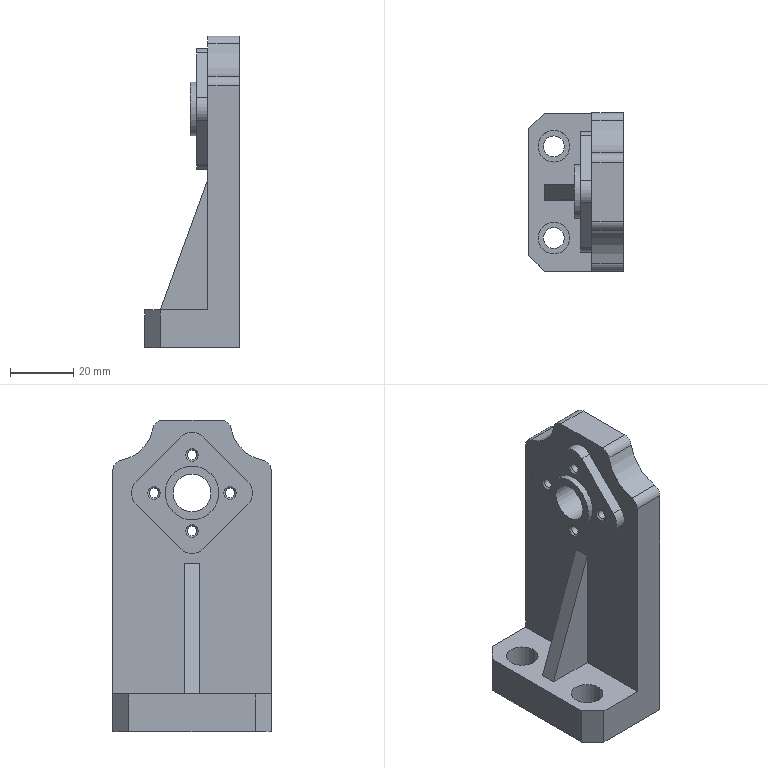Component | NX | BRACKET_A | 1 solid | 49 faces | volume 59637 mm3 | plane 21 | cylinder 20 | cone 8 | commonest cylinder face diameters 10 x6 6 x4 3 x4 26 x2 6.6 x2 17 x1 12 x1